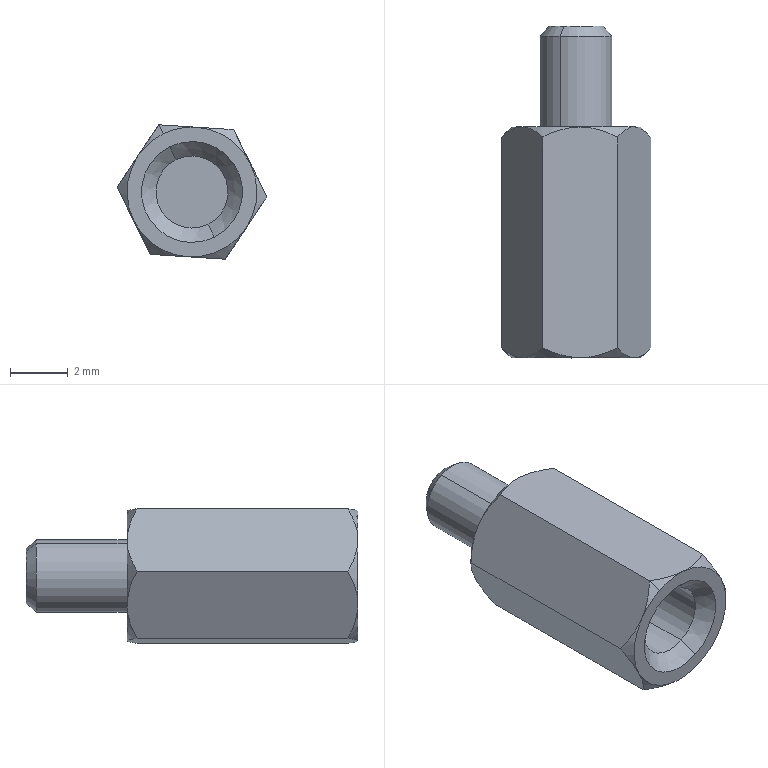Component | SolidWorks | 8.Piller-1 | 1 solid | 32 faces | box 5.19 x 11.5 x 4.66 mm | volume 132 mm3 | cone 18 | plane 10 | cylinder 4 | commonest cylinder face diameters 2.5 x4
STEP:
#1=COLOUR_RGB('',0.7922,0.8196,0.9333);
#2=FILL_AREA_STYLE_COLOUR('',#1);
#3=FILL_AREA_STYLE('',(#2));
#4=SURFACE_STYLE_FILL_AREA(#3);
#5=SURFACE_SIDE_STYLE('',(#4));
#6=SURFACE_STYLE_USAGE(.BOTH.,#5);
#7=PRESENTATION_STYLE_ASSIGNMENT((#6));
#8=CARTESIAN_POINT('',(-2.514,-0.1378,2.742));
#9=VERTEX_POINT('',#8);
#10=CARTESIAN_POINT('',(-2.558,-0.1378,2.83));
#11=VERTEX_POINT('',#10);
#12=CARTESIAN_POINT('',(-2.536,-0.1378,2.786));
#13=DIRECTION('',(0.,-1.,-0.));
#14=DIRECTION('',(-0.4434,0.,0.8963));
#15=AXIS2_PLACEMENT_3D('',#12,#13,#14);
#16=CIRCLE('',#15,0.04921);
#17=EDGE_CURVE('',#9,#11,#16,.T.);
#18=ORIENTED_EDGE('',*,*,#17,.F.);
#19=CARTESIAN_POINT('',(-2.505,-0.1575,2.725));
#20=VERTEX_POINT('',#19);
#21=CARTESIAN_POINT('',(-2.514,-0.1378,2.742));
#22=DIRECTION('',(0.3135,-0.7071,-0.6338));
#23=VECTOR('',#22,39.37);
#24=LINE('',#21,#23);
#25=EDGE_CURVE('',#9,#20,#24,.T.);
#26=ORIENTED_EDGE('',*,*,#25,.T.);
#27=CARTESIAN_POINT('',(-2.566,-0.1575,2.848));
#28=VERTEX_POINT('',#27);
#29=CARTESIAN_POINT('',(-2.536,-0.1575,2.786));
#30=DIRECTION('',(-0.,1.,0.));
#31=DIRECTION('',(-0.4434,0.,0.8963));
#32=AXIS2_PLACEMENT_3D('',#29,#30,#31);
#33=CIRCLE('',#32,0.0689);
#34=EDGE_CURVE('',#28,#20,#33,.T.);
#35=ORIENTED_EDGE('',*,*,#34,.F.);
#36=CARTESIAN_POINT('',(-2.558,-0.1378,2.83));
#37=DIRECTION('',(-0.3135,-0.7071,0.6338));
#38=VECTOR('',#37,39.37);
#39=LINE('',#36,#38);
#40=EDGE_CURVE('',#11,#28,#39,.T.);
#41=ORIENTED_EDGE('',*,*,#40,.F.);
#42=EDGE_LOOP('',(#18,#26,#35,#41));
#43=FACE_OUTER_BOUND('',#42,.T.);
#44=CARTESIAN_POINT('',(-2.536,-0.1378,2.786));
#45=DIRECTION('',(0.,-1.,-0.));
#46=DIRECTION('',(-0.4434,0.,0.8963));
#47=AXIS2_PLACEMENT_3D('',#44,#45,#46);
#48=CONICAL_SURFACE('',#47,0.04921,0.7854);
#49=ADVANCED_FACE('',(#43),#48,.F.);
#50=CARTESIAN_POINT('',(-2.519,0.2953,2.753));
#51=VERTEX_POINT('',#50);
#52=CARTESIAN_POINT('',(-2.552,0.2953,2.82));
#53=VERTEX_POINT('',#52);
#54=CARTESIAN_POINT('',(-2.536,0.2953,2.786));
#55=DIRECTION('',(-0.,1.,0.));
#56=DIRECTION('',(-0.4434,0.,0.8963));
#57=AXIS2_PLACEMENT_3D('',#54,#55,#56);
#58=CIRCLE('',#57,0.0374);
#59=EDGE_CURVE('',#51,#53,#58,.T.);
#60=ORIENTED_EDGE('',*,*,#59,.F.);
#61=CARTESIAN_POINT('',(-2.514,0.2812,2.742));
#62=VERTEX_POINT('',#61);
#63=CARTESIAN_POINT('',(-2.514,0.2812,2.742));
#64=DIRECTION('',(0.285,-0.766,-0.5762));
#65=VECTOR('',#64,39.37);
#66=LINE('',#63,#65);
#67=EDGE_CURVE('',#51,#62,#66,.T.);
#68=ORIENTED_EDGE('',*,*,#67,.T.);
#69=CARTESIAN_POINT('',(-2.558,0.2812,2.83));
#70=VERTEX_POINT('',#69);
#71=CARTESIAN_POINT('',(-2.536,0.2812,2.786));
#72=DIRECTION('',(0.,-1.,-0.));
#73=DIRECTION('',(-0.4434,0.,0.8963));
#74=AXIS2_PLACEMENT_3D('',#71,#72,#73);
#75=CIRCLE('',#74,0.04921);
#76=EDGE_CURVE('',#70,#62,#75,.T.);
#77=ORIENTED_EDGE('',*,*,#76,.F.);
#78=CARTESIAN_POINT('',(-2.558,0.2812,2.83));
#79=DIRECTION('',(-0.285,-0.766,0.5762));
#80=VECTOR('',#79,39.37);
#81=LINE('',#78,#80);
#82=EDGE_CURVE('',#53,#70,#81,.T.);
#83=ORIENTED_EDGE('',*,*,#82,.F.);
#84=EDGE_LOOP('',(#60,#68,#77,#83));
#85=FACE_OUTER_BOUND('',#84,.T.);
#86=CARTESIAN_POINT('',(-2.536,0.2812,2.786));
#87=DIRECTION('',(0.,-1.,-0.));
#88=DIRECTION('',(-0.4434,0.,0.8963));
#89=AXIS2_PLACEMENT_3D('',#86,#87,#88);
#90=CONICAL_SURFACE('',#89,0.04921,0.6981);
#91=ADVANCED_FACE('',(#85),#90,.T.);
#92=CARTESIAN_POINT('',(-2.558,0.1575,2.83));
#93=VERTEX_POINT('',#92);
#94=CARTESIAN_POINT('',(-2.514,0.1575,2.742));
#95=VERTEX_POINT('',#94);
#96=CARTESIAN_POINT('',(-2.536,0.1575,2.786));
#97=DIRECTION('',(0.,-1.,-0.));
#98=DIRECTION('',(-0.4434,0.,0.8963));
#99=AXIS2_PLACEMENT_3D('',#96,#97,#98);
#100=CIRCLE('',#99,0.04921);
#101=EDGE_CURVE('',#93,#95,#100,.T.);
#102=ORIENTED_EDGE('',*,*,#101,.F.);
#103=CARTESIAN_POINT('',(-2.558,0.1575,2.83));
#104=DIRECTION('',(-0.,1.,0.));
#105=VECTOR('',#104,39.37);
#106=LINE('',#103,#105);
#107=EDGE_CURVE('',#93,#70,#106,.T.);
#108=ORIENTED_EDGE('',*,*,#107,.T.);
#109=ORIENTED_EDGE('',*,*,#76,.T.);
#110=CARTESIAN_POINT('',(-2.514,0.1575,2.742));
#111=DIRECTION('',(-0.,1.,0.));
#112=VECTOR('',#111,39.37);
#113=LINE('',#110,#112);
#114=EDGE_CURVE('',#95,#62,#113,.T.);
#115=ORIENTED_EDGE('',*,*,#114,.F.);
#116=EDGE_LOOP('',(#102,#108,#109,#115));
#117=FACE_OUTER_BOUND('',#116,.T.);
#118=CARTESIAN_POINT('',(-2.536,0.1575,2.786));
#119=DIRECTION('',(-0.,1.,0.));
#120=DIRECTION('',(0.4434,0.,-0.8963));
#121=AXIS2_PLACEMENT_3D('',#118,#119,#120);
#122=CYLINDRICAL_SURFACE('',#121,0.04921);
#123=ADVANCED_FACE('',(#117),#122,.T.);
#124=CARTESIAN_POINT('',(-2.541,0.1575,2.698));
#125=VERTEX_POINT('',#124);
#126=CARTESIAN_POINT('',(-2.496,0.1575,2.707));
#127=VERTEX_POINT('',#126);
#128=CARTESIAN_POINT('',(-2.536,0.1575,2.786));
#129=DIRECTION('',(0.,-1.,-0.));
#130=DIRECTION('',(-0.4434,0.,0.8963));
#131=AXIS2_PLACEMENT_3D('',#128,#129,#130);
#132=CIRCLE('',#131,0.08858);
#133=EDGE_CURVE('',#125,#127,#132,.T.);
#134=ORIENTED_EDGE('',*,*,#133,.T.);
#135=CARTESIAN_POINT('',(-2.49,0.1438,2.695));
#136=VERTEX_POINT('',#135);
#137=CARTESIAN_POINT('',(-2.496,0.1575,2.707));
#138=DIRECTION('',(0.3135,-0.7071,-0.6338));
#139=VECTOR('',#138,39.37);
#140=LINE('',#137,#139);
#141=EDGE_CURVE('',#127,#136,#140,.T.);
#142=ORIENTED_EDGE('',*,*,#141,.T.);
#143=CARTESIAN_POINT('',(-2.49,0.1438,2.695));
#144=CARTESIAN_POINT('',(-2.498,0.1478,2.695));
#145=CARTESIAN_POINT('',(-2.507,0.1512,2.696));
#146=CARTESIAN_POINT('',(-2.519,0.1548,2.696));
#147=CARTESIAN_POINT('',(-2.524,0.1558,2.697));
#148=CARTESIAN_POINT('',(-2.532,0.1571,2.697));
#149=CARTESIAN_POINT('',(-2.537,0.1575,2.698));
#150=CARTESIAN_POINT('',(-2.541,0.1575,2.698));
#151=B_SPLINE_CURVE_WITH_KNOTS('',3,(#143,#144,#145,#146,#147,#148,#149,#150),.UNSPECIFIED.,.F.,.F.,(4,2,2,4),(0.00000025,0.0006735,0.00101,0.001347),.UNSPECIFIED.);
#152=EDGE_CURVE('',#136,#125,#151,.T.);
#153=ORIENTED_EDGE('',*,*,#152,.T.);
#154=EDGE_LOOP('',(#134,#142,#153));
#155=FACE_OUTER_BOUND('',#154,.T.);
#156=CARTESIAN_POINT('',(-2.536,0.1575,2.786));
#157=DIRECTION('',(0.,-1.,-0.));
#158=DIRECTION('',(0.4434,0.,-0.8963));
#159=AXIS2_PLACEMENT_3D('',#156,#157,#158);
#160=CONICAL_SURFACE('',#159,0.08858,0.7854);
#161=ADVANCED_FACE('',(#155),#160,.T.);
#162=CARTESIAN_POINT('',(-2.514,0.0315,2.742));
#163=VERTEX_POINT('',#162);
#164=CARTESIAN_POINT('',(-2.558,0.0315,2.83));
#165=VERTEX_POINT('',#164);
#166=CARTESIAN_POINT('',(-2.536,0.0315,2.786));
#167=DIRECTION('',(0.,-1.,-0.));
#168=DIRECTION('',(-0.4434,0.,0.8963));
#169=AXIS2_PLACEMENT_3D('',#166,#167,#168);
#170=CIRCLE('',#169,0.04921);
#171=EDGE_CURVE('',#163,#165,#170,.T.);
#172=ORIENTED_EDGE('',*,*,#171,.F.);
#173=CARTESIAN_POINT('',(-2.514,0.0315,2.742));
#174=DIRECTION('',(0.,-1.,-0.));
#175=VECTOR('',#174,39.37);
#176=LINE('',#173,#175);
#177=EDGE_CURVE('',#163,#9,#176,.T.);
#178=ORIENTED_EDGE('',*,*,#177,.T.);
#179=ORIENTED_EDGE('',*,*,#17,.T.);
#180=CARTESIAN_POINT('',(-2.558,0.0315,2.83));
#181=DIRECTION('',(0.,-1.,-0.));
#182=VECTOR('',#181,39.37);
#183=LINE('',#180,#182);
#184=EDGE_CURVE('',#165,#11,#183,.T.);
#185=ORIENTED_EDGE('',*,*,#184,.F.);
#186=EDGE_LOOP('',(#172,#178,#179,#185));
#187=FACE_OUTER_BOUND('',#186,.T.);
#188=CARTESIAN_POINT('',(-2.536,0.0315,2.786));
#189=DIRECTION('',(0.,-1.,-0.));
#190=DIRECTION('',(-0.4434,0.,0.8963));
#191=AXIS2_PLACEMENT_3D('',#188,#189,#190);
#192=CYLINDRICAL_SURFACE('',#191,0.04921);
#193=ADVANCED_FACE('',(#187),#192,.F.);
#194=CARTESIAN_POINT('',(-2.575,-0.1575,2.866));
#195=VERTEX_POINT('',#194);
#196=CARTESIAN_POINT('',(-2.609,-0.1575,2.835));
#197=VERTEX_POINT('',#196);
#198=CARTESIAN_POINT('',(-2.536,-0.1575,2.786));
#199=DIRECTION('',(0.,-1.,-0.));
#200=DIRECTION('',(-0.4434,0.,0.8963));
#201=AXIS2_PLACEMENT_3D('',#198,#199,#200);
#202=CIRCLE('',#201,0.08858);
#203=EDGE_CURVE('',#195,#197,#202,.T.);
#204=ORIENTED_EDGE('',*,*,#203,.F.);
#205=CARTESIAN_POINT('',(-2.581,-0.1438,2.878));
#206=VERTEX_POINT('',#205);
#207=CARTESIAN_POINT('',(-2.575,-0.1575,2.866));
#208=DIRECTION('',(-0.3135,0.7071,0.6338));
#209=VECTOR('',#208,39.37);
#210=LINE('',#207,#209);
#211=EDGE_CURVE('',#195,#206,#210,.T.);
#212=ORIENTED_EDGE('',*,*,#211,.T.);
#213=CARTESIAN_POINT('',(-2.581,-0.1438,2.878));
#214=CARTESIAN_POINT('',(-2.586,-0.1478,2.871));
#215=CARTESIAN_POINT('',(-2.59,-0.1512,2.864));
#216=CARTESIAN_POINT('',(-2.597,-0.1548,2.854));
#217=CARTESIAN_POINT('',(-2.6,-0.1558,2.85));
#218=CARTESIAN_POINT('',(-2.604,-0.1571,2.843));
#219=CARTESIAN_POINT('',(-2.607,-0.1575,2.839));
#220=CARTESIAN_POINT('',(-2.609,-0.1575,2.835));
#221=B_SPLINE_CURVE_WITH_KNOTS('',3,(#213,#214,#215,#216,#217,#218,#219,#220),.UNSPECIFIED.,.F.,.F.,(4,2,2,4),(0.00000025,0.0006735,0.00101,0.001347),.UNSPECIFIED.);
#222=EDGE_CURVE('',#206,#197,#221,.T.);
#223=ORIENTED_EDGE('',*,*,#222,.T.);
#224=EDGE_LOOP('',(#204,#212,#223));
#225=FACE_OUTER_BOUND('',#224,.T.);
#226=CARTESIAN_POINT('',(-2.536,-0.1575,2.786));
#227=DIRECTION('',(-0.,1.,0.));
#228=DIRECTION('',(-0.4434,0.,0.8963));
#229=AXIS2_PLACEMENT_3D('',#226,#227,#228);
#230=CONICAL_SURFACE('',#229,0.08858,0.7854);
#231=ADVANCED_FACE('',(#225),#230,.T.);
#232=CARTESIAN_POINT('',(-2.592,0.1438,2.701));
#233=VERTEX_POINT('',#232);
#234=CARTESIAN_POINT('',(-2.615,0.1575,2.747));
#235=VERTEX_POINT('',#234);
#236=CARTESIAN_POINT('',(-2.592,0.1438,2.701));
#237=CARTESIAN_POINT('',(-2.596,0.1477,2.708));
#238=CARTESIAN_POINT('',(-2.6,0.1511,2.716));
#239=CARTESIAN_POINT('',(-2.607,0.1561,2.731));
#240=CARTESIAN_POINT('',(-2.611,0.1575,2.739));
#241=CARTESIAN_POINT('',(-2.615,0.1575,2.747));
#242=B_SPLINE_CURVE_WITH_KNOTS('',3,(#236,#237,#238,#239,#240,#241),.UNSPECIFIED.,.F.,.F.,(4,2,4),(0.007878,0.008549,0.00922),.UNSPECIFIED.);
#243=EDGE_CURVE('',#233,#235,#242,.T.);
#244=ORIENTED_EDGE('',*,*,#243,.F.);
#245=CARTESIAN_POINT('',(-2.592,-0.1438,2.701));
#246=VERTEX_POINT('',#245);
#247=CARTESIAN_POINT('',(-2.592,-0.1575,2.701));
#248=DIRECTION('',(-0.,1.,0.));
#249=VECTOR('',#248,39.37);
#250=LINE('',#247,#249);
#251=EDGE_CURVE('',#246,#233,#250,.T.);
#252=ORIENTED_EDGE('',*,*,#251,.F.);
#253=CARTESIAN_POINT('',(-2.615,-0.1575,2.747));
#254=VERTEX_POINT('',#253);
#255=CARTESIAN_POINT('',(-2.615,-0.1575,2.747));
#256=CARTESIAN_POINT('',(-2.611,-0.1575,2.739));
#257=CARTESIAN_POINT('',(-2.607,-0.1561,2.731));
#258=CARTESIAN_POINT('',(-2.6,-0.1512,2.716));
#259=CARTESIAN_POINT('',(-2.596,-0.1477,2.708));
#260=CARTESIAN_POINT('',(-2.592,-0.1438,2.701));
#261=B_SPLINE_CURVE_WITH_KNOTS('',3,(#255,#256,#257,#258,#259,#260),.UNSPECIFIED.,.F.,.F.,(4,2,4),(0.01003,0.0107,0.01138),.UNSPECIFIED.);
#262=EDGE_CURVE('',#254,#246,#261,.T.);
#263=ORIENTED_EDGE('',*,*,#262,.F.);
#264=CARTESIAN_POINT('',(-2.638,-0.1438,2.793));
#265=VERTEX_POINT('',#264);
#266=CARTESIAN_POINT('',(-2.638,-0.1438,2.793));
#267=CARTESIAN_POINT('',(-2.634,-0.1477,2.786));
#268=CARTESIAN_POINT('',(-2.631,-0.1512,2.778));
#269=CARTESIAN_POINT('',(-2.623,-0.1561,2.763));
#270=CARTESIAN_POINT('',(-2.619,-0.1575,2.755));
#271=CARTESIAN_POINT('',(-2.615,-0.1575,2.747));
#272=B_SPLINE_CURVE_WITH_KNOTS('',3,(#266,#267,#268,#269,#270,#271),.UNSPECIFIED.,.F.,.F.,(4,2,4),(0.008681,0.009356,0.01003),.UNSPECIFIED.);
#273=EDGE_CURVE('',#265,#254,#272,.T.);
#274=ORIENTED_EDGE('',*,*,#273,.F.);
#275=CARTESIAN_POINT('',(-2.638,0.1438,2.793));
#276=VERTEX_POINT('',#275);
#277=CARTESIAN_POINT('',(-2.638,-0.1575,2.793));
#278=DIRECTION('',(-0.,1.,0.));
#279=VECTOR('',#278,39.37);
#280=LINE('',#277,#279);
#281=EDGE_CURVE('',#265,#276,#280,.T.);
#282=ORIENTED_EDGE('',*,*,#281,.T.);
#283=CARTESIAN_POINT('',(-2.615,0.1575,2.747));
#284=CARTESIAN_POINT('',(-2.619,0.1575,2.755));
#285=CARTESIAN_POINT('',(-2.623,0.1561,2.763));
#286=CARTESIAN_POINT('',(-2.631,0.1512,2.778));
#287=CARTESIAN_POINT('',(-2.634,0.1477,2.786));
#288=CARTESIAN_POINT('',(-2.638,0.1438,2.793));
#289=B_SPLINE_CURVE_WITH_KNOTS('',3,(#283,#284,#285,#286,#287,#288),.UNSPECIFIED.,.F.,.F.,(4,2,4),(0.00922,0.009892,0.01056),.UNSPECIFIED.);
#290=EDGE_CURVE('',#235,#276,#289,.T.);
#291=ORIENTED_EDGE('',*,*,#290,.F.);
#292=EDGE_LOOP('',(#244,#252,#263,#274,#282,#291));
#293=FACE_OUTER_BOUND('',#292,.T.);
#294=CARTESIAN_POINT('',(-2.638,-0.1575,2.793));
#295=DIRECTION('',(0.8963,-0.,0.4434));
#296=DIRECTION('',(-0.4434,-0.,0.8963));
#297=AXIS2_PLACEMENT_3D('',#294,#295,#296);
#298=PLANE('',#297);
#299=ADVANCED_FACE('',(#293),#298,.F.);
#300=ORIENTED_EDGE('',*,*,#152,.F.);
#301=CARTESIAN_POINT('',(-2.49,-0.1438,2.695));
#302=VERTEX_POINT('',#301);
#303=CARTESIAN_POINT('',(-2.49,-0.1575,2.695));
#304=DIRECTION('',(-0.,1.,0.));
#305=VECTOR('',#304,39.37);
#306=LINE('',#303,#305);
#307=EDGE_CURVE('',#302,#136,#306,.T.);
#308=ORIENTED_EDGE('',*,*,#307,.F.);
#309=CARTESIAN_POINT('',(-2.541,-0.1575,2.698));
#310=VERTEX_POINT('',#309);
#311=CARTESIAN_POINT('',(-2.541,-0.1575,2.698));
#312=CARTESIAN_POINT('',(-2.533,-0.1575,2.697));
#313=CARTESIAN_POINT('',(-2.524,-0.1561,2.697));
#314=CARTESIAN_POINT('',(-2.507,-0.1512,2.696));
#315=CARTESIAN_POINT('',(-2.498,-0.1478,2.695));
#316=CARTESIAN_POINT('',(-2.49,-0.1438,2.695));
#317=B_SPLINE_CURVE_WITH_KNOTS('',3,(#311,#312,#313,#314,#315,#316),.UNSPECIFIED.,.F.,.F.,(4,2,4),(0.001347,0.002015,0.002684),.UNSPECIFIED.);
#318=EDGE_CURVE('',#310,#302,#317,.T.);
#319=ORIENTED_EDGE('',*,*,#318,.F.);
#320=CARTESIAN_POINT('',(-2.592,-0.1438,2.701));
#321=CARTESIAN_POINT('',(-2.584,-0.1478,2.701));
#322=CARTESIAN_POINT('',(-2.576,-0.1512,2.7));
#323=CARTESIAN_POINT('',(-2.564,-0.1548,2.699));
#324=CARTESIAN_POINT('',(-2.559,-0.1558,2.699));
#325=CARTESIAN_POINT('',(-2.55,-0.1571,2.698));
#326=CARTESIAN_POINT('',(-2.546,-0.1575,2.698));
#327=CARTESIAN_POINT('',(-2.541,-0.1575,2.698));
#328=B_SPLINE_CURVE_WITH_KNOTS('',3,(#320,#321,#322,#323,#324,#325,#326,#327),.UNSPECIFIED.,.F.,.F.,(4,2,2,4),(0.00000025,0.0006735,0.00101,0.001347),.UNSPECIFIED.);
#329=EDGE_CURVE('',#246,#310,#328,.T.);
#330=ORIENTED_EDGE('',*,*,#329,.F.);
#331=ORIENTED_EDGE('',*,*,#251,.T.);
#332=CARTESIAN_POINT('',(-2.541,0.1575,2.698));
#333=CARTESIAN_POINT('',(-2.55,0.1575,2.698));
#334=CARTESIAN_POINT('',(-2.559,0.1561,2.699));
#335=CARTESIAN_POINT('',(-2.576,0.1512,2.7));
#336=CARTESIAN_POINT('',(-2.584,0.1478,2.701));
#337=CARTESIAN_POINT('',(-2.592,0.1438,2.701));
#338=B_SPLINE_CURVE_WITH_KNOTS('',3,(#332,#333,#334,#335,#336,#337),.UNSPECIFIED.,.F.,.F.,(4,2,4),(0.001347,0.002015,0.002684),.UNSPECIFIED.);
#339=EDGE_CURVE('',#125,#233,#338,.T.);
#340=ORIENTED_EDGE('',*,*,#339,.F.);
#341=EDGE_LOOP('',(#300,#308,#319,#330,#331,#340));
#342=FACE_OUTER_BOUND('',#341,.T.);
#343=CARTESIAN_POINT('',(-2.592,-0.1575,2.701));
#344=DIRECTION('',(0.0642,-0.,0.9979));
#345=DIRECTION('',(-0.9979,-0.,0.0642));
#346=AXIS2_PLACEMENT_3D('',#343,#344,#345);
#347=PLANE('',#346);
#348=ADVANCED_FACE('',(#342),#347,.F.);
#349=CARTESIAN_POINT('',(-2.434,0.1438,2.78));
#350=VERTEX_POINT('',#349);
#351=CARTESIAN_POINT('',(-2.462,0.1575,2.737));
#352=VERTEX_POINT('',#351);
#353=CARTESIAN_POINT('',(-2.434,0.1438,2.78));
#354=CARTESIAN_POINT('',(-2.438,0.1478,2.773));
#355=CARTESIAN_POINT('',(-2.443,0.1512,2.766));
#356=CARTESIAN_POINT('',(-2.45,0.1548,2.756));
#357=CARTESIAN_POINT('',(-2.452,0.1558,2.752));
#358=CARTESIAN_POINT('',(-2.457,0.1571,2.745));
#359=CARTESIAN_POINT('',(-2.46,0.1575,2.741));
#360=CARTESIAN_POINT('',(-2.462,0.1575,2.737));
#361=B_SPLINE_CURVE_WITH_KNOTS('',3,(#353,#354,#355,#356,#357,#358,#359,#360),.UNSPECIFIED.,.F.,.F.,(4,2,2,4),(0.00000025,0.0006735,0.00101,0.001347),.UNSPECIFIED.);
#362=EDGE_CURVE('',#350,#352,#361,.T.);
#363=ORIENTED_EDGE('',*,*,#362,.F.);
#364=CARTESIAN_POINT('',(-2.434,-0.1438,2.78));
#365=VERTEX_POINT('',#364);
#366=CARTESIAN_POINT('',(-2.434,-0.1575,2.78));
#367=DIRECTION('',(-0.,1.,0.));
#368=VECTOR('',#367,39.37);
#369=LINE('',#366,#368);
#370=EDGE_CURVE('',#365,#350,#369,.T.);
#371=ORIENTED_EDGE('',*,*,#370,.F.);
#372=CARTESIAN_POINT('',(-2.462,-0.1575,2.737));
#373=VERTEX_POINT('',#372);
#374=CARTESIAN_POINT('',(-2.462,-0.1575,2.737));
#375=CARTESIAN_POINT('',(-2.457,-0.1575,2.745));
#376=CARTESIAN_POINT('',(-2.452,-0.1561,2.752));
#377=CARTESIAN_POINT('',(-2.443,-0.1512,2.766));
#378=CARTESIAN_POINT('',(-2.438,-0.1478,2.773));
#379=CARTESIAN_POINT('',(-2.434,-0.1438,2.78));
#380=B_SPLINE_CURVE_WITH_KNOTS('',3,(#374,#375,#376,#377,#378,#379),.UNSPECIFIED.,.F.,.F.,(4,2,4),(0.001347,0.002015,0.002684),.UNSPECIFIED.);
#381=EDGE_CURVE('',#373,#365,#380,.T.);
#382=ORIENTED_EDGE('',*,*,#381,.F.);
#383=CARTESIAN_POINT('',(-2.49,-0.1438,2.695));
#384=CARTESIAN_POINT('',(-2.486,-0.1478,2.701));
#385=CARTESIAN_POINT('',(-2.481,-0.1512,2.708));
#386=CARTESIAN_POINT('',(-2.474,-0.1548,2.719));
#387=CARTESIAN_POINT('',(-2.472,-0.1558,2.722));
#388=CARTESIAN_POINT('',(-2.467,-0.1571,2.73));
#389=CARTESIAN_POINT('',(-2.464,-0.1575,2.733));
#390=CARTESIAN_POINT('',(-2.462,-0.1575,2.737));
#391=B_SPLINE_CURVE_WITH_KNOTS('',3,(#383,#384,#385,#386,#387,#388,#389,#390),.UNSPECIFIED.,.F.,.F.,(4,2,2,4),(0.00000025,0.0006735,0.00101,0.001347),.UNSPECIFIED.);
#392=EDGE_CURVE('',#302,#373,#391,.T.);
#393=ORIENTED_EDGE('',*,*,#392,.F.);
#394=ORIENTED_EDGE('',*,*,#307,.T.);
#395=CARTESIAN_POINT('',(-2.462,0.1575,2.737));
#396=CARTESIAN_POINT('',(-2.467,0.1575,2.73));
#397=CARTESIAN_POINT('',(-2.472,0.1561,2.722));
#398=CARTESIAN_POINT('',(-2.481,0.1512,2.708));
#399=CARTESIAN_POINT('',(-2.486,0.1478,2.701));
#400=CARTESIAN_POINT('',(-2.49,0.1438,2.695));
#401=B_SPLINE_CURVE_WITH_KNOTS('',3,(#395,#396,#397,#398,#399,#400),.UNSPECIFIED.,.F.,.F.,(4,2,4),(0.001347,0.002015,0.002684),.UNSPECIFIED.);
#402=EDGE_CURVE('',#352,#136,#401,.T.);
#403=ORIENTED_EDGE('',*,*,#402,.F.);
#404=EDGE_LOOP('',(#363,#371,#382,#393,#394,#403));
#405=FACE_OUTER_BOUND('',#404,.T.);
#406=CARTESIAN_POINT('',(-2.49,-0.1575,2.695));
#407=DIRECTION('',(-0.8321,-0.,0.5546));
#408=DIRECTION('',(-0.5546,0.,-0.8321));
#409=AXIS2_PLACEMENT_3D('',#406,#407,#408);
#410=PLANE('',#409);
#411=ADVANCED_FACE('',(#405),#410,.F.);
#412=CARTESIAN_POINT('',(-2.479,0.1438,2.871));
#413=VERTEX_POINT('',#412);
#414=CARTESIAN_POINT('',(-2.456,0.1575,2.826));
#415=VERTEX_POINT('',#414);
#416=CARTESIAN_POINT('',(-2.479,0.1438,2.871));
#417=CARTESIAN_POINT('',(-2.475,0.1477,2.864));
#418=CARTESIAN_POINT('',(-2.472,0.1512,2.857));
#419=CARTESIAN_POINT('',(-2.464,0.1561,2.841));
#420=CARTESIAN_POINT('',(-2.46,0.1575,2.834));
#421=CARTESIAN_POINT('',(-2.456,0.1575,2.826));
#422=B_SPLINE_CURVE_WITH_KNOTS('',3,(#416,#417,#418,#419,#420,#421),.UNSPECIFIED.,.F.,.F.,(4,2,4),(0.00895,0.009624,0.0103),.UNSPECIFIED.);
#423=EDGE_CURVE('',#413,#415,#422,.T.);
#424=ORIENTED_EDGE('',*,*,#423,.F.);
#425=CARTESIAN_POINT('',(-2.479,-0.1438,2.871));
#426=VERTEX_POINT('',#425);
#427=CARTESIAN_POINT('',(-2.479,-0.1575,2.871));
#428=DIRECTION('',(-0.,1.,0.));
#429=VECTOR('',#428,39.37);
#430=LINE('',#427,#429);
#431=EDGE_CURVE('',#426,#413,#430,.T.);
#432=ORIENTED_EDGE('',*,*,#431,.F.);
#433=CARTESIAN_POINT('',(-2.456,-0.1575,2.826));
#434=VERTEX_POINT('',#433);
#435=CARTESIAN_POINT('',(-2.456,-0.1575,2.826));
#436=CARTESIAN_POINT('',(-2.46,-0.1575,2.834));
#437=CARTESIAN_POINT('',(-2.464,-0.1561,2.841));
#438=CARTESIAN_POINT('',(-2.472,-0.1512,2.857));
#439=CARTESIAN_POINT('',(-2.475,-0.1477,2.864));
#440=CARTESIAN_POINT('',(-2.479,-0.1438,2.871));
#441=B_SPLINE_CURVE_WITH_KNOTS('',3,(#435,#436,#437,#438,#439,#440),.UNSPECIFIED.,.F.,.F.,(4,2,4),(0.009638,0.01031,0.01098),.UNSPECIFIED.);
#442=EDGE_CURVE('',#434,#426,#441,.T.);
#443=ORIENTED_EDGE('',*,*,#442,.F.);
#444=CARTESIAN_POINT('',(-2.434,-0.1438,2.78));
#445=CARTESIAN_POINT('',(-2.437,-0.1477,2.787));
#446=CARTESIAN_POINT('',(-2.441,-0.1512,2.794));
#447=CARTESIAN_POINT('',(-2.448,-0.1561,2.81));
#448=CARTESIAN_POINT('',(-2.452,-0.1575,2.818));
#449=CARTESIAN_POINT('',(-2.456,-0.1575,2.826));
#450=B_SPLINE_CURVE_WITH_KNOTS('',3,(#444,#445,#446,#447,#448,#449),.UNSPECIFIED.,.F.,.F.,(4,2,4),(0.008296,0.008967,0.009638),.UNSPECIFIED.);
#451=EDGE_CURVE('',#365,#434,#450,.T.);
#452=ORIENTED_EDGE('',*,*,#451,.F.);
#453=ORIENTED_EDGE('',*,*,#370,.T.);
#454=CARTESIAN_POINT('',(-2.456,0.1575,2.826));
#455=CARTESIAN_POINT('',(-2.452,0.1575,2.817));
#456=CARTESIAN_POINT('',(-2.448,0.1561,2.81));
#457=CARTESIAN_POINT('',(-2.441,0.1511,2.794));
#458=CARTESIAN_POINT('',(-2.437,0.1477,2.787));
#459=CARTESIAN_POINT('',(-2.434,0.1438,2.78));
#460=B_SPLINE_CURVE_WITH_KNOTS('',3,(#454,#455,#456,#457,#458,#459),.UNSPECIFIED.,.F.,.F.,(4,2,4),(0.0103,0.01097,0.01165),.UNSPECIFIED.);
#461=EDGE_CURVE('',#415,#350,#460,.T.);
#462=ORIENTED_EDGE('',*,*,#461,.F.);
#463=EDGE_LOOP('',(#424,#432,#443,#452,#453,#462));
#464=FACE_OUTER_BOUND('',#463,.T.);
#465=CARTESIAN_POINT('',(-2.434,-0.1575,2.78));
#466=DIRECTION('',(-0.8963,0.,-0.4434));
#467=DIRECTION('',(0.4434,0.,-0.8963));
#468=AXIS2_PLACEMENT_3D('',#465,#466,#467);
#469=PLANE('',#468);
#470=ADVANCED_FACE('',(#464),#469,.F.);
#471=CARTESIAN_POINT('',(-2.581,0.1438,2.878));
#472=VERTEX_POINT('',#471);
#473=CARTESIAN_POINT('',(-2.53,0.1575,2.875));
#474=VERTEX_POINT('',#473);
#475=CARTESIAN_POINT('',(-2.581,0.1438,2.878));
#476=CARTESIAN_POINT('',(-2.573,0.1478,2.877));
#477=CARTESIAN_POINT('',(-2.565,0.1512,2.877));
#478=CARTESIAN_POINT('',(-2.552,0.1548,2.876));
#479=CARTESIAN_POINT('',(-2.548,0.1558,2.876));
#480=CARTESIAN_POINT('',(-2.539,0.1571,2.875));
#481=CARTESIAN_POINT('',(-2.534,0.1575,2.875));
#482=CARTESIAN_POINT('',(-2.53,0.1575,2.875));
#483=B_SPLINE_CURVE_WITH_KNOTS('',3,(#475,#476,#477,#478,#479,#480,#481,#482),.UNSPECIFIED.,.F.,.F.,(4,2,2,4),(0.00000025,0.0006735,0.00101,0.001347),.UNSPECIFIED.);
#484=EDGE_CURVE('',#472,#474,#483,.T.);
#485=ORIENTED_EDGE('',*,*,#484,.F.);
#486=CARTESIAN_POINT('',(-2.581,-0.1575,2.878));
#487=DIRECTION('',(-0.,1.,0.));
#488=VECTOR('',#487,39.37);
#489=LINE('',#486,#488);
#490=EDGE_CURVE('',#206,#472,#489,.T.);
#491=ORIENTED_EDGE('',*,*,#490,.F.);
#492=CARTESIAN_POINT('',(-2.53,-0.1575,2.875));
#493=VERTEX_POINT('',#492);
#494=CARTESIAN_POINT('',(-2.53,-0.1575,2.875));
#495=CARTESIAN_POINT('',(-2.539,-0.1575,2.875));
#496=CARTESIAN_POINT('',(-2.548,-0.1561,2.876));
#497=CARTESIAN_POINT('',(-2.565,-0.1512,2.877));
#498=CARTESIAN_POINT('',(-2.573,-0.1478,2.877));
#499=CARTESIAN_POINT('',(-2.581,-0.1438,2.878));
#500=B_SPLINE_CURVE_WITH_KNOTS('',3,(#494,#495,#496,#497,#498,#499),.UNSPECIFIED.,.F.,.F.,(4,2,4),(0.001347,0.002015,0.002684),.UNSPECIFIED.);
#501=EDGE_CURVE('',#493,#206,#500,.T.);
#502=ORIENTED_EDGE('',*,*,#501,.F.);
#503=CARTESIAN_POINT('',(-2.479,-0.1438,2.871));
#504=CARTESIAN_POINT('',(-2.487,-0.1478,2.872));
#505=CARTESIAN_POINT('',(-2.495,-0.1512,2.872));
#506=CARTESIAN_POINT('',(-2.508,-0.1548,2.873));
#507=CARTESIAN_POINT('',(-2.512,-0.1558,2.874));
#508=CARTESIAN_POINT('',(-2.521,-0.1571,2.874));
#509=CARTESIAN_POINT('',(-2.526,-0.1575,2.874));
#510=CARTESIAN_POINT('',(-2.53,-0.1575,2.875));
#511=B_SPLINE_CURVE_WITH_KNOTS('',3,(#503,#504,#505,#506,#507,#508,#509,#510),.UNSPECIFIED.,.F.,.F.,(4,2,2,4),(0.00000025,0.0006735,0.00101,0.001347),.UNSPECIFIED.);
#512=EDGE_CURVE('',#426,#493,#511,.T.);
#513=ORIENTED_EDGE('',*,*,#512,.F.);
#514=ORIENTED_EDGE('',*,*,#431,.T.);
#515=CARTESIAN_POINT('',(-2.53,0.1575,2.875));
#516=CARTESIAN_POINT('',(-2.521,0.1575,2.874));
#517=CARTESIAN_POINT('',(-2.512,0.1561,2.874));
#518=CARTESIAN_POINT('',(-2.495,0.1512,2.872));
#519=CARTESIAN_POINT('',(-2.487,0.1478,2.872));
#520=CARTESIAN_POINT('',(-2.479,0.1438,2.871));
#521=B_SPLINE_CURVE_WITH_KNOTS('',3,(#515,#516,#517,#518,#519,#520),.UNSPECIFIED.,.F.,.F.,(4,2,4),(0.001347,0.002015,0.002684),.UNSPECIFIED.);
#522=EDGE_CURVE('',#474,#413,#521,.T.);
#523=ORIENTED_EDGE('',*,*,#522,.F.);
#524=EDGE_LOOP('',(#485,#491,#502,#513,#514,#523));
#525=FACE_OUTER_BOUND('',#524,.T.);
#526=CARTESIAN_POINT('',(-2.479,-0.1575,2.871));
#527=DIRECTION('',(-0.0642,0.,-0.9979));
#528=DIRECTION('',(0.9979,0.,-0.0642));
#529=AXIS2_PLACEMENT_3D('',#526,#527,#528);
#530=PLANE('',#529);
#531=ADVANCED_FACE('',(#525),#530,.F.);
#532=CARTESIAN_POINT('',(-2.609,0.1575,2.835));
#533=VERTEX_POINT('',#532);
#534=CARTESIAN_POINT('',(-2.638,0.1438,2.793));
#535=CARTESIAN_POINT('',(-2.633,0.1478,2.8));
#536=CARTESIAN_POINT('',(-2.629,0.1512,2.806));
#537=CARTESIAN_POINT('',(-2.622,0.1548,2.817));
#538=CARTESIAN_POINT('',(-2.619,0.1558,2.821));
#539=CARTESIAN_POINT('',(-2.614,0.1571,2.828));
#540=CARTESIAN_POINT('',(-2.612,0.1575,2.832));
#541=CARTESIAN_POINT('',(-2.609,0.1575,2.835));
#542=B_SPLINE_CURVE_WITH_KNOTS('',3,(#534,#535,#536,#537,#538,#539,#540,#541),.UNSPECIFIED.,.F.,.F.,(4,2,2,4),(0.00000025,0.0006735,0.00101,0.001347),.UNSPECIFIED.);
#543=EDGE_CURVE('',#276,#533,#542,.T.);
#544=ORIENTED_EDGE('',*,*,#543,.F.);
#545=ORIENTED_EDGE('',*,*,#281,.F.);
#546=CARTESIAN_POINT('',(-2.609,-0.1575,2.835));
#547=CARTESIAN_POINT('',(-2.614,-0.1575,2.828));
#548=CARTESIAN_POINT('',(-2.619,-0.1561,2.821));
#549=CARTESIAN_POINT('',(-2.629,-0.1512,2.806));
#550=CARTESIAN_POINT('',(-2.633,-0.1478,2.799));
#551=CARTESIAN_POINT('',(-2.638,-0.1438,2.793));
#552=B_SPLINE_CURVE_WITH_KNOTS('',3,(#546,#547,#548,#549,#550,#551),.UNSPECIFIED.,.F.,.F.,(4,2,4),(0.001347,0.002015,0.002684),.UNSPECIFIED.);
#553=EDGE_CURVE('',#197,#265,#552,.T.);
#554=ORIENTED_EDGE('',*,*,#553,.F.);
#555=ORIENTED_EDGE('',*,*,#222,.F.);
#556=ORIENTED_EDGE('',*,*,#490,.T.);
#557=CARTESIAN_POINT('',(-2.609,0.1575,2.835));
#558=CARTESIAN_POINT('',(-2.604,0.1575,2.843));
#559=CARTESIAN_POINT('',(-2.6,0.1561,2.85));
#560=CARTESIAN_POINT('',(-2.59,0.1512,2.864));
#561=CARTESIAN_POINT('',(-2.586,0.1478,2.871));
#562=CARTESIAN_POINT('',(-2.581,0.1438,2.878));
#563=B_SPLINE_CURVE_WITH_KNOTS('',3,(#557,#558,#559,#560,#561,#562),.UNSPECIFIED.,.F.,.F.,(4,2,4),(0.001347,0.002015,0.002684),.UNSPECIFIED.);
#564=EDGE_CURVE('',#533,#472,#563,.T.);
#565=ORIENTED_EDGE('',*,*,#564,.F.);
#566=EDGE_LOOP('',(#544,#545,#554,#555,#556,#565));
#567=FACE_OUTER_BOUND('',#566,.T.);
#568=CARTESIAN_POINT('',(-2.581,-0.1575,2.878));
#569=DIRECTION('',(0.8321,0.,-0.5546));
#570=DIRECTION('',(0.5546,-0.,0.8321));
#571=AXIS2_PLACEMENT_3D('',#568,#569,#570);
#572=PLANE('',#571);
#573=ADVANCED_FACE('',(#567),#572,.F.);
#574=ORIENTED_EDGE('',*,*,#211,.F.);
#575=CARTESIAN_POINT('',(-2.536,-0.1575,2.786));
#576=DIRECTION('',(0.,-1.,-0.));
#577=DIRECTION('',(-0.4434,0.,0.8963));
#578=AXIS2_PLACEMENT_3D('',#575,#576,#577);
#579=CIRCLE('',#578,0.08858);
#580=EDGE_CURVE('',#493,#195,#579,.T.);
#581=ORIENTED_EDGE('',*,*,#580,.F.);
#582=ORIENTED_EDGE('',*,*,#501,.T.);
#583=EDGE_LOOP('',(#574,#581,#582));
#584=FACE_OUTER_BOUND('',#583,.T.);
#585=CARTESIAN_POINT('',(-2.536,-0.1575,2.786));
#586=DIRECTION('',(-0.,1.,0.));
#587=DIRECTION('',(-0.4434,0.,0.8963));
#588=AXIS2_PLACEMENT_3D('',#585,#586,#587);
#589=CONICAL_SURFACE('',#588,0.08858,0.7854);
#590=ADVANCED_FACE('',(#584),#589,.T.);
#591=ORIENTED_EDGE('',*,*,#442,.T.);
#592=ORIENTED_EDGE('',*,*,#512,.T.);
#593=CARTESIAN_POINT('',(-2.536,-0.1575,2.786));
#594=DIRECTION('',(0.,-1.,-0.));
#595=DIRECTION('',(-0.4434,0.,0.8963));
#596=AXIS2_PLACEMENT_3D('',#593,#594,#595);
#597=CIRCLE('',#596,0.08858);
#598=EDGE_CURVE('',#434,#493,#597,.T.);
#599=ORIENTED_EDGE('',*,*,#598,.F.);
#600=EDGE_LOOP('',(#591,#592,#599));
#601=FACE_OUTER_BOUND('',#600,.T.);
#602=CARTESIAN_POINT('',(-2.536,-0.1575,2.786));
#603=DIRECTION('',(-0.,1.,0.));
#604=DIRECTION('',(-0.4434,0.,0.8963));
#605=AXIS2_PLACEMENT_3D('',#602,#603,#604);
#606=CONICAL_SURFACE('',#605,0.08858,0.7854);
#607=ADVANCED_FACE('',(#601),#606,.T.);
#608=ORIENTED_EDGE('',*,*,#381,.T.);
#609=ORIENTED_EDGE('',*,*,#451,.T.);
#610=CARTESIAN_POINT('',(-2.536,-0.1575,2.786));
#611=DIRECTION('',(0.,-1.,-0.));
#612=DIRECTION('',(-0.4434,0.,0.8963));
#613=AXIS2_PLACEMENT_3D('',#610,#611,#612);
#614=CIRCLE('',#613,0.08858);
#615=EDGE_CURVE('',#373,#434,#614,.T.);
#616=ORIENTED_EDGE('',*,*,#615,.F.);
#617=EDGE_LOOP('',(#608,#609,#616));
#618=FACE_OUTER_BOUND('',#617,.T.);
#619=CARTESIAN_POINT('',(-2.536,-0.1575,2.786));
#620=DIRECTION('',(-0.,1.,0.));
#621=DIRECTION('',(-0.4434,0.,0.8963));
#622=AXIS2_PLACEMENT_3D('',#619,#620,#621);
#623=CONICAL_SURFACE('',#622,0.08858,0.7854);
#624=ADVANCED_FACE('',(#618),#623,.T.);
#625=ORIENTED_EDGE('',*,*,#318,.T.);
#626=ORIENTED_EDGE('',*,*,#392,.T.);
#627=CARTESIAN_POINT('',(-2.536,-0.1575,2.786));
#628=DIRECTION('',(0.,-1.,-0.));
#629=DIRECTION('',(-0.4434,0.,0.8963));
#630=AXIS2_PLACEMENT_3D('',#627,#628,#629);
#631=CIRCLE('',#630,0.08858);
#632=EDGE_CURVE('',#310,#373,#631,.T.);
#633=ORIENTED_EDGE('',*,*,#632,.F.);
#634=EDGE_LOOP('',(#625,#626,#633));
#635=FACE_OUTER_BOUND('',#634,.T.);
#636=CARTESIAN_POINT('',(-2.536,-0.1575,2.786));
#637=DIRECTION('',(-0.,1.,0.));
#638=DIRECTION('',(-0.4434,0.,0.8963));
#639=AXIS2_PLACEMENT_3D('',#636,#637,#638);
#640=CONICAL_SURFACE('',#639,0.08858,0.7854);
#641=ADVANCED_FACE('',(#635),#640,.T.);
#642=ORIENTED_EDGE('',*,*,#262,.T.);
#643=ORIENTED_EDGE('',*,*,#329,.T.);
#644=CARTESIAN_POINT('',(-2.536,-0.1575,2.786));
#645=DIRECTION('',(0.,-1.,-0.));
#646=DIRECTION('',(-0.4434,0.,0.8963));
#647=AXIS2_PLACEMENT_3D('',#644,#645,#646);
#648=CIRCLE('',#647,0.08858);
#649=EDGE_CURVE('',#254,#310,#648,.T.);
#650=ORIENTED_EDGE('',*,*,#649,.F.);
#651=EDGE_LOOP('',(#642,#643,#650));
#652=FACE_OUTER_BOUND('',#651,.T.);
#653=CARTESIAN_POINT('',(-2.536,-0.1575,2.786));
#654=DIRECTION('',(-0.,1.,0.));
#655=DIRECTION('',(-0.4434,0.,0.8963));
#656=AXIS2_PLACEMENT_3D('',#653,#654,#655);
#657=CONICAL_SURFACE('',#656,0.08858,0.7854);
#658=ADVANCED_FACE('',(#652),#657,.T.);
#659=ORIENTED_EDGE('',*,*,#273,.T.);
#660=CARTESIAN_POINT('',(-2.536,-0.1575,2.786));
#661=DIRECTION('',(0.,-1.,-0.));
#662=DIRECTION('',(-0.4434,0.,0.8963));
#663=AXIS2_PLACEMENT_3D('',#660,#661,#662);
#664=CIRCLE('',#663,0.08858);
#665=EDGE_CURVE('',#197,#254,#664,.T.);
#666=ORIENTED_EDGE('',*,*,#665,.F.);
#667=ORIENTED_EDGE('',*,*,#553,.T.);
#668=EDGE_LOOP('',(#659,#666,#667));
#669=FACE_OUTER_BOUND('',#668,.T.);
#670=CARTESIAN_POINT('',(-2.536,-0.1575,2.786));
#671=DIRECTION('',(-0.,1.,0.));
#672=DIRECTION('',(-0.4434,0.,0.8963));
#673=AXIS2_PLACEMENT_3D('',#670,#671,#672);
#674=CONICAL_SURFACE('',#673,0.08858,0.7854);
#675=ADVANCED_FACE('',(#669),#674,.T.);
#676=CARTESIAN_POINT('',(-2.536,0.0315,2.786));
#677=DIRECTION('',(0.,-1.,-0.));
#678=DIRECTION('',(-0.4434,0.,0.8963));
#679=AXIS2_PLACEMENT_3D('',#676,#677,#678);
#680=CIRCLE('',#679,0.04921);
#681=EDGE_CURVE('',#165,#163,#680,.T.);
#682=ORIENTED_EDGE('',*,*,#681,.T.);
#683=ORIENTED_EDGE('',*,*,#171,.T.);
#684=EDGE_LOOP('',(#682,#683));
#685=FACE_OUTER_BOUND('',#684,.T.);
#686=CARTESIAN_POINT('',(-2.536,0.0315,2.786));
#687=DIRECTION('',(0.,-1.,-0.));
#688=DIRECTION('',(-0.4434,-0.,0.8963));
#689=AXIS2_PLACEMENT_3D('',#686,#687,#688);
#690=PLANE('',#689);
#691=ADVANCED_FACE('',(#685),#690,.T.);
#692=ORIENTED_EDGE('',*,*,#177,.F.);
#693=ORIENTED_EDGE('',*,*,#681,.F.);
#694=ORIENTED_EDGE('',*,*,#184,.T.);
#695=CARTESIAN_POINT('',(-2.536,-0.1378,2.786));
#696=DIRECTION('',(0.,-1.,-0.));
#697=DIRECTION('',(-0.4434,0.,0.8963));
#698=AXIS2_PLACEMENT_3D('',#695,#696,#697);
#699=CIRCLE('',#698,0.04921);
#700=EDGE_CURVE('',#11,#9,#699,.T.);
#701=ORIENTED_EDGE('',*,*,#700,.T.);
#702=EDGE_LOOP('',(#692,#693,#694,#701));
#703=FACE_OUTER_BOUND('',#702,.T.);
#704=CARTESIAN_POINT('',(-2.536,0.0315,2.786));
#705=DIRECTION('',(0.,-1.,-0.));
#706=DIRECTION('',(-0.4434,0.,0.8963));
#707=AXIS2_PLACEMENT_3D('',#704,#705,#706);
#708=CYLINDRICAL_SURFACE('',#707,0.04921);
#709=ADVANCED_FACE('',(#703),#708,.F.);
#710=ORIENTED_EDGE('',*,*,#34,.T.);
#711=CARTESIAN_POINT('',(-2.536,-0.1575,2.786));
#712=DIRECTION('',(-0.,1.,0.));
#713=DIRECTION('',(-0.4434,0.,0.8963));
#714=AXIS2_PLACEMENT_3D('',#711,#712,#713);
#715=CIRCLE('',#714,0.0689);
#716=EDGE_CURVE('',#20,#28,#715,.T.);
#717=ORIENTED_EDGE('',*,*,#716,.T.);
#718=EDGE_LOOP('',(#710,#717));
#719=FACE_BOUND('',#718,.T.);
#720=ORIENTED_EDGE('',*,*,#580,.T.);
#721=ORIENTED_EDGE('',*,*,#203,.T.);
#722=ORIENTED_EDGE('',*,*,#665,.T.);
#723=ORIENTED_EDGE('',*,*,#649,.T.);
#724=ORIENTED_EDGE('',*,*,#632,.T.);
#725=ORIENTED_EDGE('',*,*,#615,.T.);
#726=ORIENTED_EDGE('',*,*,#598,.T.);
#727=EDGE_LOOP('',(#720,#721,#722,#723,#724,#725,#726));
#728=FACE_OUTER_BOUND('',#727,.T.);
#729=CARTESIAN_POINT('',(-2.536,-0.1575,2.786));
#730=DIRECTION('',(0.,-1.,-0.));
#731=DIRECTION('',(-0.4434,-0.,0.8963));
#732=AXIS2_PLACEMENT_3D('',#729,#730,#731);
#733=PLANE('',#732);
#734=ADVANCED_FACE('',(#719,#728),#733,.T.);
#735=ORIENTED_EDGE('',*,*,#484,.T.);
#736=CARTESIAN_POINT('',(-2.536,0.1575,2.786));
#737=DIRECTION('',(0.,-1.,-0.));
#738=DIRECTION('',(-0.4434,0.,0.8963));
#739=AXIS2_PLACEMENT_3D('',#736,#737,#738);
#740=CIRCLE('',#739,0.08858);
#741=EDGE_CURVE('',#474,#533,#740,.T.);
#742=ORIENTED_EDGE('',*,*,#741,.T.);
#743=ORIENTED_EDGE('',*,*,#564,.T.);
#744=EDGE_LOOP('',(#735,#742,#743));
#745=FACE_OUTER_BOUND('',#744,.T.);
#746=CARTESIAN_POINT('',(-2.536,0.1575,2.786));
#747=DIRECTION('',(0.,-1.,-0.));
#748=DIRECTION('',(0.4434,0.,-0.8963));
#749=AXIS2_PLACEMENT_3D('',#746,#747,#748);
#750=CONICAL_SURFACE('',#749,0.08858,0.7854);
#751=ADVANCED_FACE('',(#745),#750,.T.);
#752=ORIENTED_EDGE('',*,*,#423,.T.);
#753=CARTESIAN_POINT('',(-2.536,0.1575,2.786));
#754=DIRECTION('',(0.,-1.,-0.));
#755=DIRECTION('',(-0.4434,0.,0.8963));
#756=AXIS2_PLACEMENT_3D('',#753,#754,#755);
#757=CIRCLE('',#756,0.08858);
#758=EDGE_CURVE('',#415,#474,#757,.T.);
#759=ORIENTED_EDGE('',*,*,#758,.T.);
#760=ORIENTED_EDGE('',*,*,#522,.T.);
#761=EDGE_LOOP('',(#752,#759,#760));
#762=FACE_OUTER_BOUND('',#761,.T.);
#763=CARTESIAN_POINT('',(-2.536,0.1575,2.786));
#764=DIRECTION('',(0.,-1.,-0.));
#765=DIRECTION('',(0.4434,0.,-0.8963));
#766=AXIS2_PLACEMENT_3D('',#763,#764,#765);
#767=CONICAL_SURFACE('',#766,0.08858,0.7854);
#768=ADVANCED_FACE('',(#762),#767,.T.);
#769=ORIENTED_EDGE('',*,*,#362,.T.);
#770=CARTESIAN_POINT('',(-2.536,0.1575,2.786));
#771=DIRECTION('',(0.,-1.,-0.));
#772=DIRECTION('',(-0.4434,0.,0.8963));
#773=AXIS2_PLACEMENT_3D('',#770,#771,#772);
#774=CIRCLE('',#773,0.08858);
#775=EDGE_CURVE('',#352,#415,#774,.T.);
#776=ORIENTED_EDGE('',*,*,#775,.T.);
#777=ORIENTED_EDGE('',*,*,#461,.T.);
#778=EDGE_LOOP('',(#769,#776,#777));
#779=FACE_OUTER_BOUND('',#778,.T.);
#780=CARTESIAN_POINT('',(-2.536,0.1575,2.786));
#781=DIRECTION('',(0.,-1.,-0.));
#782=DIRECTION('',(0.4434,0.,-0.8963));
#783=AXIS2_PLACEMENT_3D('',#780,#781,#782);
#784=CONICAL_SURFACE('',#783,0.08858,0.7854);
#785=ADVANCED_FACE('',(#779),#784,.T.);
#786=ORIENTED_EDGE('',*,*,#141,.F.);
#787=CARTESIAN_POINT('',(-2.536,0.1575,2.786));
#788=DIRECTION('',(0.,-1.,-0.));
#789=DIRECTION('',(-0.4434,0.,0.8963));
#790=AXIS2_PLACEMENT_3D('',#787,#788,#789);
#791=CIRCLE('',#790,0.08858);
#792=EDGE_CURVE('',#127,#352,#791,.T.);
#793=ORIENTED_EDGE('',*,*,#792,.T.);
#794=ORIENTED_EDGE('',*,*,#402,.T.);
#795=EDGE_LOOP('',(#786,#793,#794));
#796=FACE_OUTER_BOUND('',#795,.T.);
#797=CARTESIAN_POINT('',(-2.536,0.1575,2.786));
#798=DIRECTION('',(0.,-1.,-0.));
#799=DIRECTION('',(0.4434,0.,-0.8963));
#800=AXIS2_PLACEMENT_3D('',#797,#798,#799);
#801=CONICAL_SURFACE('',#800,0.08858,0.7854);
#802=ADVANCED_FACE('',(#796),#801,.T.);
#803=ORIENTED_EDGE('',*,*,#339,.T.);
#804=ORIENTED_EDGE('',*,*,#243,.T.);
#805=CARTESIAN_POINT('',(-2.536,0.1575,2.786));
#806=DIRECTION('',(-0.,1.,0.));
#807=DIRECTION('',(0.4434,0.,-0.8963));
#808=AXIS2_PLACEMENT_3D('',#805,#806,#807);
#809=CIRCLE('',#808,0.08858);
#810=EDGE_CURVE('',#125,#235,#809,.T.);
#811=ORIENTED_EDGE('',*,*,#810,.F.);
#812=EDGE_LOOP('',(#803,#804,#811));
#813=FACE_OUTER_BOUND('',#812,.T.);
#814=CARTESIAN_POINT('',(-2.536,0.1575,2.786));
#815=DIRECTION('',(0.,-1.,-0.));
#816=DIRECTION('',(0.4434,0.,-0.8963));
#817=AXIS2_PLACEMENT_3D('',#814,#815,#816);
#818=CONICAL_SURFACE('',#817,0.08858,0.7854);
#819=ADVANCED_FACE('',(#813),#818,.T.);
#820=ORIENTED_EDGE('',*,*,#290,.T.);
#821=ORIENTED_EDGE('',*,*,#543,.T.);
#822=CARTESIAN_POINT('',(-2.536,0.1575,2.786));
#823=DIRECTION('',(0.,-1.,-0.));
#824=DIRECTION('',(-0.4434,0.,0.8963));
#825=AXIS2_PLACEMENT_3D('',#822,#823,#824);
#826=CIRCLE('',#825,0.08858);
#827=EDGE_CURVE('',#533,#235,#826,.T.);
#828=ORIENTED_EDGE('',*,*,#827,.T.);
#829=EDGE_LOOP('',(#820,#821,#828));
#830=FACE_OUTER_BOUND('',#829,.T.);
#831=CARTESIAN_POINT('',(-2.536,0.1575,2.786));
#832=DIRECTION('',(0.,-1.,-0.));
#833=DIRECTION('',(0.4434,0.,-0.8963));
#834=AXIS2_PLACEMENT_3D('',#831,#832,#833);
#835=CONICAL_SURFACE('',#834,0.08858,0.7854);
#836=ADVANCED_FACE('',(#830),#835,.T.);
#837=CARTESIAN_POINT('',(-2.536,0.2953,2.786));
#838=DIRECTION('',(-0.,1.,0.));
#839=DIRECTION('',(-0.4434,0.,0.8963));
#840=AXIS2_PLACEMENT_3D('',#837,#838,#839);
#841=CIRCLE('',#840,0.0374);
#842=EDGE_CURVE('',#53,#51,#841,.T.);
#843=ORIENTED_EDGE('',*,*,#842,.T.);
#844=ORIENTED_EDGE('',*,*,#59,.T.);
#845=EDGE_LOOP('',(#843,#844));
#846=FACE_OUTER_BOUND('',#845,.T.);
#847=CARTESIAN_POINT('',(-2.536,0.2953,2.786));
#848=DIRECTION('',(0.,-1.,-0.));
#849=DIRECTION('',(-0.4434,-0.,0.8963));
#850=AXIS2_PLACEMENT_3D('',#847,#848,#849);
#851=PLANE('',#850);
#852=ADVANCED_FACE('',(#846),#851,.F.);
#853=ORIENTED_EDGE('',*,*,#107,.F.);
#854=CARTESIAN_POINT('',(-2.536,0.1575,2.786));
#855=DIRECTION('',(0.,-1.,-0.));
#856=DIRECTION('',(-0.4434,0.,0.8963));
#857=AXIS2_PLACEMENT_3D('',#854,#855,#856);
#858=CIRCLE('',#857,0.04921);
#859=EDGE_CURVE('',#95,#93,#858,.T.);
#860=ORIENTED_EDGE('',*,*,#859,.F.);
#861=ORIENTED_EDGE('',*,*,#114,.T.);
#862=CARTESIAN_POINT('',(-2.536,0.2812,2.786));
#863=DIRECTION('',(0.,-1.,-0.));
#864=DIRECTION('',(-0.4434,0.,0.8963));
#865=AXIS2_PLACEMENT_3D('',#862,#863,#864);
#866=CIRCLE('',#865,0.04921);
#867=EDGE_CURVE('',#62,#70,#866,.T.);
#868=ORIENTED_EDGE('',*,*,#867,.T.);
#869=EDGE_LOOP('',(#853,#860,#861,#868));
#870=FACE_OUTER_BOUND('',#869,.T.);
#871=CARTESIAN_POINT('',(-2.536,0.1575,2.786));
#872=DIRECTION('',(-0.,1.,0.));
#873=DIRECTION('',(0.4434,0.,-0.8963));
#874=AXIS2_PLACEMENT_3D('',#871,#872,#873);
#875=CYLINDRICAL_SURFACE('',#874,0.04921);
#876=ADVANCED_FACE('',(#870),#875,.T.);
#877=ORIENTED_EDGE('',*,*,#859,.T.);
#878=ORIENTED_EDGE('',*,*,#101,.T.);
#879=EDGE_LOOP('',(#877,#878));
#880=FACE_BOUND('',#879,.T.);
#881=ORIENTED_EDGE('',*,*,#827,.F.);
#882=ORIENTED_EDGE('',*,*,#741,.F.);
#883=ORIENTED_EDGE('',*,*,#758,.F.);
#884=ORIENTED_EDGE('',*,*,#775,.F.);
#885=ORIENTED_EDGE('',*,*,#792,.F.);
#886=ORIENTED_EDGE('',*,*,#133,.F.);
#887=ORIENTED_EDGE('',*,*,#810,.T.);
#888=EDGE_LOOP('',(#881,#882,#883,#884,#885,#886,#887));
#889=FACE_OUTER_BOUND('',#888,.T.);
#890=CARTESIAN_POINT('',(-2.536,0.1575,2.786));
#891=DIRECTION('',(0.,-1.,-0.));
#892=DIRECTION('',(-0.4434,-0.,0.8963));
#893=AXIS2_PLACEMENT_3D('',#890,#891,#892);
#894=PLANE('',#893);
#895=ADVANCED_FACE('',(#880,#889),#894,.F.);
#896=ORIENTED_EDGE('',*,*,#67,.F.);
#897=ORIENTED_EDGE('',*,*,#842,.F.);
#898=ORIENTED_EDGE('',*,*,#82,.T.);
#899=ORIENTED_EDGE('',*,*,#867,.F.);
#900=EDGE_LOOP('',(#896,#897,#898,#899));
#901=FACE_OUTER_BOUND('',#900,.T.);
#902=CARTESIAN_POINT('',(-2.536,0.2812,2.786));
#903=DIRECTION('',(0.,-1.,-0.));
#904=DIRECTION('',(-0.4434,0.,0.8963));
#905=AXIS2_PLACEMENT_3D('',#902,#903,#904);
#906=CONICAL_SURFACE('',#905,0.04921,0.6981);
#907=ADVANCED_FACE('',(#901),#906,.T.);
#908=ORIENTED_EDGE('',*,*,#25,.F.);
#909=ORIENTED_EDGE('',*,*,#700,.F.);
#910=ORIENTED_EDGE('',*,*,#40,.T.);
#911=ORIENTED_EDGE('',*,*,#716,.F.);
#912=EDGE_LOOP('',(#908,#909,#910,#911));
#913=FACE_OUTER_BOUND('',#912,.T.);
#914=CARTESIAN_POINT('',(-2.536,-0.1378,2.786));
#915=DIRECTION('',(0.,-1.,-0.));
#916=DIRECTION('',(-0.4434,0.,0.8963));
#917=AXIS2_PLACEMENT_3D('',#914,#915,#916);
#918=CONICAL_SURFACE('',#917,0.04921,0.7854);
#919=ADVANCED_FACE('',(#913),#918,.F.);
#920=CLOSED_SHELL('',(#49,#91,#123,#161,#193,#231,#299,#348,#411,#470,#531,#573,#590,#607,#624,#641,#658,#675,#691,#709,#734,#751,#768,#785,#802,#819,#836,#852,#876,#895,#907,#919));
#921=MANIFOLD_SOLID_BREP('',#920);
#922=STYLED_ITEM('',(#7),#921);
#923=PRESENTATION_LAYER_ASSIGNMENT('','',(#922));
#924=(LENGTH_UNIT()NAMED_UNIT(*)SI_UNIT($,.METRE.));
#925=LENGTH_MEASURE_WITH_UNIT(LENGTH_MEASURE(0.0254),#924);
#926=DIMENSIONAL_EXPONENTS(1.,0.,0.,0.,0.,0.,0.);
#927=(CONVERSION_BASED_UNIT('',#925)LENGTH_UNIT()NAMED_UNIT(#926));
#928=UNCERTAINTY_MEASURE_WITH_UNIT(LENGTH_MEASURE(0.00001),#927,'','');
#929=(NAMED_UNIT(*)PLANE_ANGLE_UNIT()SI_UNIT($,.RADIAN.));
#930=(NAMED_UNIT(*)SI_UNIT($,.STERADIAN.)SOLID_ANGLE_UNIT());
#931=(GEOMETRIC_REPRESENTATION_CONTEXT(3)GLOBAL_UNCERTAINTY_ASSIGNED_CONTEXT((#928))GLOBAL_UNIT_ASSIGNED_CONTEXT((#927,#929,#930))REPRESENTATION_CONTEXT('',''));
#932=MECHANICAL_DESIGN_GEOMETRIC_PRESENTATION_REPRESENTATION('',(#922),#931);
#933=CARTESIAN_POINT('',(0.,0.,0.));
#934=DIRECTION('',(0.,0.,1.));
#935=DIRECTION('',(1.,0.,0.));
#936=AXIS2_PLACEMENT_3D('',#933,#934,#935);
#937=(LENGTH_UNIT()NAMED_UNIT(*)SI_UNIT($,.METRE.));
#938=LENGTH_MEASURE_WITH_UNIT(LENGTH_MEASURE(0.0254),#937);
#939=DIMENSIONAL_EXPONENTS(1.,0.,0.,0.,0.,0.,0.);
#940=(CONVERSION_BASED_UNIT('',#938)LENGTH_UNIT()NAMED_UNIT(#939));
#941=UNCERTAINTY_MEASURE_WITH_UNIT(LENGTH_MEASURE(0.00001),#940,'','');
#942=(NAMED_UNIT(*)PLANE_ANGLE_UNIT()SI_UNIT($,.RADIAN.));
#943=(NAMED_UNIT(*)SI_UNIT($,.STERADIAN.)SOLID_ANGLE_UNIT());
#944=(GEOMETRIC_REPRESENTATION_CONTEXT(3)GLOBAL_UNCERTAINTY_ASSIGNED_CONTEXT((#941))GLOBAL_UNIT_ASSIGNED_CONTEXT((#940,#942,#943))REPRESENTATION_CONTEXT('',''));
#945=ADVANCED_BREP_SHAPE_REPRESENTATION('',(#921,#936),#944);